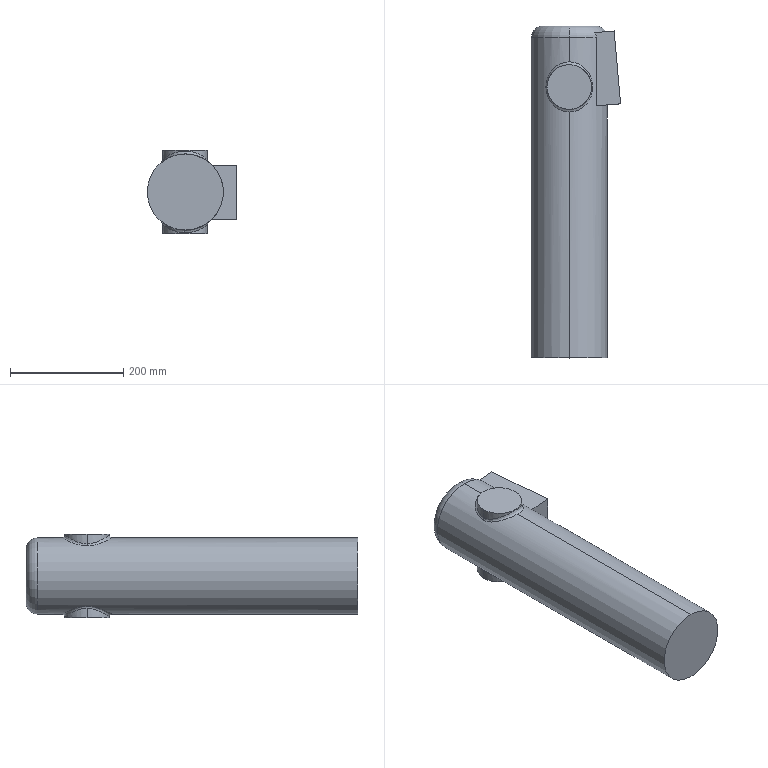Component | SolidWorks | RehabilitationChair-18-19-1 | 1 solid | 21 faces | volume 8645036 mm3 | plane 9 | cylinder 6 | spline 4 | torus 2 | commonest cylinder face diameters 78.479 x4 134.251 x2